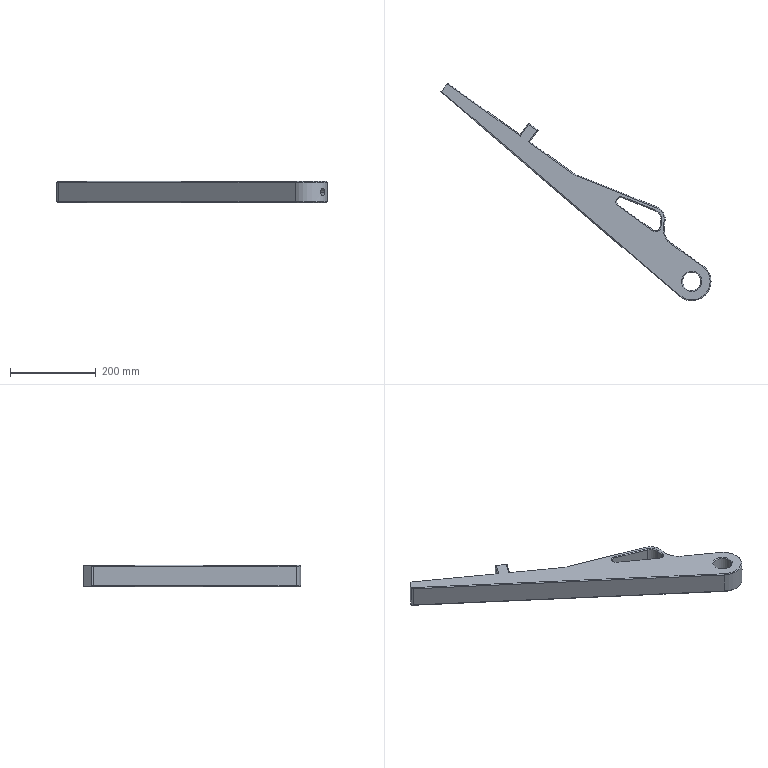Component | SolidWorks | IngotConnectingArm-2 | 1 solid | 78 faces | volume 2424689 mm3 | cylinder 37 | torus 26 | plane 15 | commonest cylinder face diameters 4 x24 16 x2 43 x2 26.366 x2 20 x2 90 x1 40.186 x1 60.186 x1 | material 45